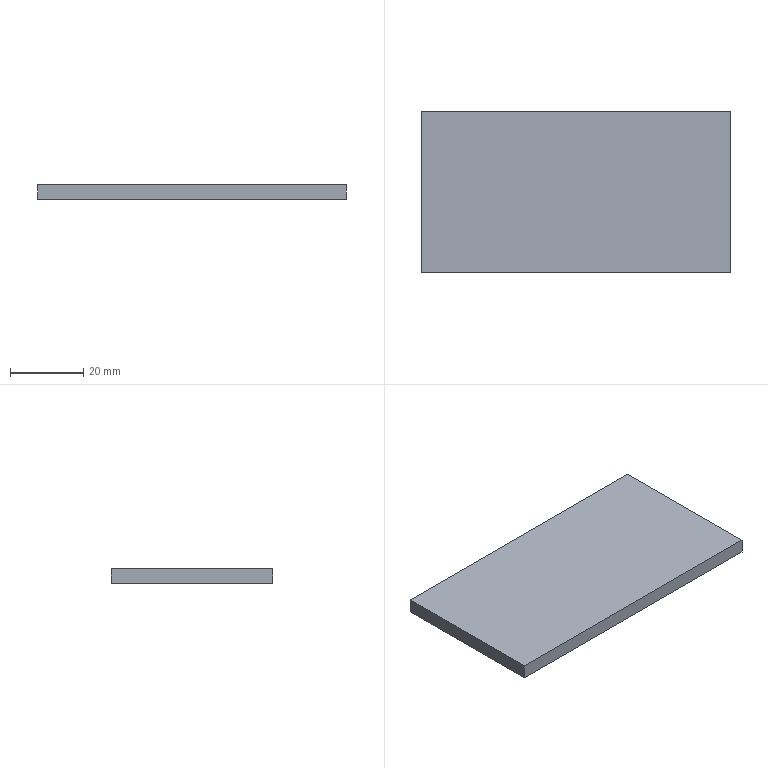Component | NX | BASE_PLATE | 1 solid | 6 faces | box 84 x 44 x 4 mm | volume 14784 mm3 | plane 6
STEP:
#1=CARTESIAN_POINT('',(0.,0.,0.));
#2=DIRECTION('',(0.,0.,1.));
#3=DIRECTION('',(1.,0.,0.));
#4=AXIS2_PLACEMENT_3D('',#1,#2,#3);
#5=CARTESIAN_POINT('',(-44.,24.,0.));
#6=VERTEX_POINT('',#5);
#7=CARTESIAN_POINT('',(-44.,-20.,0.));
#8=VERTEX_POINT('',#7);
#9=CARTESIAN_POINT('',(-44.,20.,0.));
#10=DIRECTION('',(0.,-1.,0.));
#11=VECTOR('',#10,1.);
#12=LINE('',#9,#11);
#13=CARTESIAN_POINT('',(-44.,20.,4.));
#14=DIRECTION('',(1.,0.,0.));
#15=DIRECTION('',(0.,0.,-1.));
#16=AXIS2_PLACEMENT_3D('',#13,#14,#15);
#17=PLANE('',#16);
#18=CARTESIAN_POINT('',(4.,0.));
#19=DIRECTION('',(0.,-1.));
#20=VECTOR('',#19,1.);
#21=LINE('',#18,#20);
#22=(GEOMETRIC_REPRESENTATION_CONTEXT(2)PARAMETRIC_REPRESENTATION_CONTEXT()REPRESENTATION_CONTEXT('',''));
#23=DEFINITIONAL_REPRESENTATION('',(#21),#22);
#24=PCURVE('',#17,#23);
#25=CARTESIAN_POINT('',(0.,0.,0.));
#26=DIRECTION('',(0.,0.,1.));
#27=DIRECTION('',(1.,0.,0.));
#28=AXIS2_PLACEMENT_3D('',#25,#26,#27);
#29=PLANE('',#28);
#30=CARTESIAN_POINT('',(-44.,20.));
#31=DIRECTION('',(0.,-1.));
#32=VECTOR('',#31,1.);
#33=LINE('',#30,#32);
#34=(GEOMETRIC_REPRESENTATION_CONTEXT(2)PARAMETRIC_REPRESENTATION_CONTEXT()REPRESENTATION_CONTEXT('',''));
#35=DEFINITIONAL_REPRESENTATION('',(#33),#34);
#36=PCURVE('',#29,#35);
#37=SURFACE_CURVE('',#12,(#24,#36),.PCURVE_S1.);
#38=EDGE_CURVE('',#6,#8,#37,.T.);
#39=ORIENTED_EDGE('',*,*,#38,.T.);
#40=CARTESIAN_POINT('',(-44.,-20.,4.));
#41=VERTEX_POINT('',#40);
#42=CARTESIAN_POINT('',(-44.,-20.,4.));
#43=DIRECTION('',(0.,0.,-1.));
#44=VECTOR('',#43,1.);
#45=LINE('',#42,#44);
#46=CARTESIAN_POINT('',(0.,-40.));
#47=DIRECTION('',(1.,0.));
#48=VECTOR('',#47,1.);
#49=LINE('',#46,#48);
#50=(GEOMETRIC_REPRESENTATION_CONTEXT(2)PARAMETRIC_REPRESENTATION_CONTEXT()REPRESENTATION_CONTEXT('',''));
#51=DEFINITIONAL_REPRESENTATION('',(#49),#50);
#52=PCURVE('',#17,#51);
#53=CARTESIAN_POINT('',(-40.,-20.,4.));
#54=DIRECTION('',(-0.,1.,0.));
#55=DIRECTION('',(-1.,-0.,0.));
#56=AXIS2_PLACEMENT_3D('',#53,#54,#55);
#57=PLANE('',#56);
#58=CARTESIAN_POINT('',(4.,0.));
#59=DIRECTION('',(0.,-1.));
#60=VECTOR('',#59,1.);
#61=LINE('',#58,#60);
#62=(GEOMETRIC_REPRESENTATION_CONTEXT(2)PARAMETRIC_REPRESENTATION_CONTEXT()REPRESENTATION_CONTEXT('',''));
#63=DEFINITIONAL_REPRESENTATION('',(#61),#62);
#64=PCURVE('',#57,#63);
#65=SURFACE_CURVE('',#45,(#52,#64),.PCURVE_S1.);
#66=EDGE_CURVE('',#41,#8,#65,.T.);
#67=ORIENTED_EDGE('',*,*,#66,.F.);
#68=CARTESIAN_POINT('',(-44.,24.,4.));
#69=VERTEX_POINT('',#68);
#70=CARTESIAN_POINT('',(-44.,20.,4.));
#71=DIRECTION('',(0.,-1.,0.));
#72=VECTOR('',#71,1.);
#73=LINE('',#70,#72);
#74=CARTESIAN_POINT('',(0.,0.));
#75=DIRECTION('',(0.,-1.));
#76=VECTOR('',#75,1.);
#77=LINE('',#74,#76);
#78=(GEOMETRIC_REPRESENTATION_CONTEXT(2)PARAMETRIC_REPRESENTATION_CONTEXT()REPRESENTATION_CONTEXT('',''));
#79=DEFINITIONAL_REPRESENTATION('',(#77),#78);
#80=PCURVE('',#17,#79);
#81=CARTESIAN_POINT('',(0.,0.,4.));
#82=DIRECTION('',(0.,0.,1.));
#83=DIRECTION('',(1.,0.,0.));
#84=AXIS2_PLACEMENT_3D('',#81,#82,#83);
#85=PLANE('',#84);
#86=CARTESIAN_POINT('',(-44.,20.));
#87=DIRECTION('',(0.,-1.));
#88=VECTOR('',#87,1.);
#89=LINE('',#86,#88);
#90=(GEOMETRIC_REPRESENTATION_CONTEXT(2)PARAMETRIC_REPRESENTATION_CONTEXT()REPRESENTATION_CONTEXT('',''));
#91=DEFINITIONAL_REPRESENTATION('',(#89),#90);
#92=PCURVE('',#85,#91);
#93=SURFACE_CURVE('',#73,(#80,#92),.PCURVE_S1.);
#94=EDGE_CURVE('',#69,#41,#93,.T.);
#95=ORIENTED_EDGE('',*,*,#94,.F.);
#96=CARTESIAN_POINT('',(-44.,24.,4.));
#97=DIRECTION('',(0.,0.,-1.));
#98=VECTOR('',#97,1.);
#99=LINE('',#96,#98);
#100=CARTESIAN_POINT('',(0.,4.));
#101=DIRECTION('',(1.,0.));
#102=VECTOR('',#101,1.);
#103=LINE('',#100,#102);
#104=(GEOMETRIC_REPRESENTATION_CONTEXT(2)PARAMETRIC_REPRESENTATION_CONTEXT()REPRESENTATION_CONTEXT('',''));
#105=DEFINITIONAL_REPRESENTATION('',(#103),#104);
#106=PCURVE('',#17,#105);
#107=CARTESIAN_POINT('',(40.,24.,4.));
#108=DIRECTION('',(-0.,-1.,0.));
#109=DIRECTION('',(1.,-0.,0.));
#110=AXIS2_PLACEMENT_3D('',#107,#108,#109);
#111=PLANE('',#110);
#112=CARTESIAN_POINT('',(-84.,0.));
#113=DIRECTION('',(0.,-1.));
#114=VECTOR('',#113,1.);
#115=LINE('',#112,#114);
#116=(GEOMETRIC_REPRESENTATION_CONTEXT(2)PARAMETRIC_REPRESENTATION_CONTEXT()REPRESENTATION_CONTEXT('',''));
#117=DEFINITIONAL_REPRESENTATION('',(#115),#116);
#118=PCURVE('',#111,#117);
#119=SURFACE_CURVE('',#99,(#106,#118),.PCURVE_S1.);
#120=EDGE_CURVE('',#69,#6,#119,.T.);
#121=ORIENTED_EDGE('',*,*,#120,.T.);
#122=EDGE_LOOP('',(#39,#67,#95,#121));
#123=FACE_BOUND('',#122,.T.);
#124=ADVANCED_FACE('',(#123),#17,.F.);
#125=CARTESIAN_POINT('',(40.,-20.,0.));
#126=VERTEX_POINT('',#125);
#127=CARTESIAN_POINT('',(-40.,-20.,0.));
#128=DIRECTION('',(1.,0.,0.));
#129=VECTOR('',#128,1.);
#130=LINE('',#127,#129);
#131=CARTESIAN_POINT('',(0.,-4.));
#132=DIRECTION('',(-1.,0.));
#133=VECTOR('',#132,1.);
#134=LINE('',#131,#133);
#135=(GEOMETRIC_REPRESENTATION_CONTEXT(2)PARAMETRIC_REPRESENTATION_CONTEXT()REPRESENTATION_CONTEXT('',''));
#136=DEFINITIONAL_REPRESENTATION('',(#134),#135);
#137=PCURVE('',#57,#136);
#138=CARTESIAN_POINT('',(-40.,-20.));
#139=DIRECTION('',(1.,0.));
#140=VECTOR('',#139,1.);
#141=LINE('',#138,#140);
#142=(GEOMETRIC_REPRESENTATION_CONTEXT(2)PARAMETRIC_REPRESENTATION_CONTEXT()REPRESENTATION_CONTEXT('',''));
#143=DEFINITIONAL_REPRESENTATION('',(#141),#142);
#144=PCURVE('',#29,#143);
#145=SURFACE_CURVE('',#130,(#137,#144),.PCURVE_S1.);
#146=EDGE_CURVE('',#8,#126,#145,.T.);
#147=ORIENTED_EDGE('',*,*,#146,.T.);
#148=CARTESIAN_POINT('',(40.,-20.,4.));
#149=VERTEX_POINT('',#148);
#150=CARTESIAN_POINT('',(40.,-20.,4.));
#151=DIRECTION('',(0.,0.,-1.));
#152=VECTOR('',#151,1.);
#153=LINE('',#150,#152);
#154=CARTESIAN_POINT('',(-80.,0.));
#155=DIRECTION('',(0.,-1.));
#156=VECTOR('',#155,1.);
#157=LINE('',#154,#156);
#158=(GEOMETRIC_REPRESENTATION_CONTEXT(2)PARAMETRIC_REPRESENTATION_CONTEXT()REPRESENTATION_CONTEXT('',''));
#159=DEFINITIONAL_REPRESENTATION('',(#157),#158);
#160=PCURVE('',#57,#159);
#161=CARTESIAN_POINT('',(40.,-20.,4.));
#162=DIRECTION('',(-1.,0.,0.));
#163=DIRECTION('',(0.,0.,1.));
#164=AXIS2_PLACEMENT_3D('',#161,#162,#163);
#165=PLANE('',#164);
#166=CARTESIAN_POINT('',(0.,0.));
#167=DIRECTION('',(-1.,0.));
#168=VECTOR('',#167,1.);
#169=LINE('',#166,#168);
#170=(GEOMETRIC_REPRESENTATION_CONTEXT(2)PARAMETRIC_REPRESENTATION_CONTEXT()REPRESENTATION_CONTEXT('',''));
#171=DEFINITIONAL_REPRESENTATION('',(#169),#170);
#172=PCURVE('',#165,#171);
#173=SURFACE_CURVE('',#153,(#160,#172),.PCURVE_S1.);
#174=EDGE_CURVE('',#149,#126,#173,.T.);
#175=ORIENTED_EDGE('',*,*,#174,.F.);
#176=CARTESIAN_POINT('',(-40.,-20.,4.));
#177=DIRECTION('',(1.,0.,0.));
#178=VECTOR('',#177,1.);
#179=LINE('',#176,#178);
#180=CARTESIAN_POINT('',(0.,0.));
#181=DIRECTION('',(-1.,0.));
#182=VECTOR('',#181,1.);
#183=LINE('',#180,#182);
#184=(GEOMETRIC_REPRESENTATION_CONTEXT(2)PARAMETRIC_REPRESENTATION_CONTEXT()REPRESENTATION_CONTEXT('',''));
#185=DEFINITIONAL_REPRESENTATION('',(#183),#184);
#186=PCURVE('',#57,#185);
#187=CARTESIAN_POINT('',(-40.,-20.));
#188=DIRECTION('',(1.,0.));
#189=VECTOR('',#188,1.);
#190=LINE('',#187,#189);
#191=(GEOMETRIC_REPRESENTATION_CONTEXT(2)PARAMETRIC_REPRESENTATION_CONTEXT()REPRESENTATION_CONTEXT('',''));
#192=DEFINITIONAL_REPRESENTATION('',(#190),#191);
#193=PCURVE('',#85,#192);
#194=SURFACE_CURVE('',#179,(#186,#193),.PCURVE_S1.);
#195=EDGE_CURVE('',#41,#149,#194,.T.);
#196=ORIENTED_EDGE('',*,*,#195,.F.);
#197=ORIENTED_EDGE('',*,*,#66,.T.);
#198=EDGE_LOOP('',(#147,#175,#196,#197));
#199=FACE_BOUND('',#198,.T.);
#200=ADVANCED_FACE('',(#199),#57,.F.);
#201=CARTESIAN_POINT('',(40.,24.,0.));
#202=VERTEX_POINT('',#201);
#203=CARTESIAN_POINT('',(40.,-20.,0.));
#204=DIRECTION('',(0.,1.,0.));
#205=VECTOR('',#204,1.);
#206=LINE('',#203,#205);
#207=CARTESIAN_POINT('',(-4.,0.));
#208=DIRECTION('',(0.,1.));
#209=VECTOR('',#208,1.);
#210=LINE('',#207,#209);
#211=(GEOMETRIC_REPRESENTATION_CONTEXT(2)PARAMETRIC_REPRESENTATION_CONTEXT()REPRESENTATION_CONTEXT('',''));
#212=DEFINITIONAL_REPRESENTATION('',(#210),#211);
#213=PCURVE('',#165,#212);
#214=CARTESIAN_POINT('',(40.,-20.));
#215=DIRECTION('',(0.,1.));
#216=VECTOR('',#215,1.);
#217=LINE('',#214,#216);
#218=(GEOMETRIC_REPRESENTATION_CONTEXT(2)PARAMETRIC_REPRESENTATION_CONTEXT()REPRESENTATION_CONTEXT('',''));
#219=DEFINITIONAL_REPRESENTATION('',(#217),#218);
#220=PCURVE('',#29,#219);
#221=SURFACE_CURVE('',#206,(#213,#220),.PCURVE_S1.);
#222=EDGE_CURVE('',#126,#202,#221,.T.);
#223=ORIENTED_EDGE('',*,*,#222,.T.);
#224=CARTESIAN_POINT('',(40.,24.,4.));
#225=VERTEX_POINT('',#224);
#226=CARTESIAN_POINT('',(40.,24.,4.));
#227=DIRECTION('',(0.,0.,-1.));
#228=VECTOR('',#227,1.);
#229=LINE('',#226,#228);
#230=CARTESIAN_POINT('',(0.,44.));
#231=DIRECTION('',(-1.,0.));
#232=VECTOR('',#231,1.);
#233=LINE('',#230,#232);
#234=(GEOMETRIC_REPRESENTATION_CONTEXT(2)PARAMETRIC_REPRESENTATION_CONTEXT()REPRESENTATION_CONTEXT('',''));
#235=DEFINITIONAL_REPRESENTATION('',(#233),#234);
#236=PCURVE('',#165,#235);
#237=CARTESIAN_POINT('',(0.,0.));
#238=DIRECTION('',(0.,-1.));
#239=VECTOR('',#238,1.);
#240=LINE('',#237,#239);
#241=(GEOMETRIC_REPRESENTATION_CONTEXT(2)PARAMETRIC_REPRESENTATION_CONTEXT()REPRESENTATION_CONTEXT('',''));
#242=DEFINITIONAL_REPRESENTATION('',(#240),#241);
#243=PCURVE('',#111,#242);
#244=SURFACE_CURVE('',#229,(#236,#243),.PCURVE_S1.);
#245=EDGE_CURVE('',#225,#202,#244,.T.);
#246=ORIENTED_EDGE('',*,*,#245,.F.);
#247=CARTESIAN_POINT('',(40.,-20.,4.));
#248=DIRECTION('',(0.,1.,0.));
#249=VECTOR('',#248,1.);
#250=LINE('',#247,#249);
#251=CARTESIAN_POINT('',(0.,0.));
#252=DIRECTION('',(0.,1.));
#253=VECTOR('',#252,1.);
#254=LINE('',#251,#253);
#255=(GEOMETRIC_REPRESENTATION_CONTEXT(2)PARAMETRIC_REPRESENTATION_CONTEXT()REPRESENTATION_CONTEXT('',''));
#256=DEFINITIONAL_REPRESENTATION('',(#254),#255);
#257=PCURVE('',#165,#256);
#258=CARTESIAN_POINT('',(40.,-20.));
#259=DIRECTION('',(0.,1.));
#260=VECTOR('',#259,1.);
#261=LINE('',#258,#260);
#262=(GEOMETRIC_REPRESENTATION_CONTEXT(2)PARAMETRIC_REPRESENTATION_CONTEXT()REPRESENTATION_CONTEXT('',''));
#263=DEFINITIONAL_REPRESENTATION('',(#261),#262);
#264=PCURVE('',#85,#263);
#265=SURFACE_CURVE('',#250,(#257,#264),.PCURVE_S1.);
#266=EDGE_CURVE('',#149,#225,#265,.T.);
#267=ORIENTED_EDGE('',*,*,#266,.F.);
#268=ORIENTED_EDGE('',*,*,#174,.T.);
#269=EDGE_LOOP('',(#223,#246,#267,#268));
#270=FACE_BOUND('',#269,.T.);
#271=ADVANCED_FACE('',(#270),#165,.F.);
#272=CARTESIAN_POINT('',(40.,24.,0.));
#273=DIRECTION('',(-1.,0.,0.));
#274=VECTOR('',#273,1.);
#275=LINE('',#272,#274);
#276=CARTESIAN_POINT('',(0.,-4.));
#277=DIRECTION('',(-1.,0.));
#278=VECTOR('',#277,1.);
#279=LINE('',#276,#278);
#280=(GEOMETRIC_REPRESENTATION_CONTEXT(2)PARAMETRIC_REPRESENTATION_CONTEXT()REPRESENTATION_CONTEXT('',''));
#281=DEFINITIONAL_REPRESENTATION('',(#279),#280);
#282=PCURVE('',#111,#281);
#283=CARTESIAN_POINT('',(40.,24.));
#284=DIRECTION('',(-1.,0.));
#285=VECTOR('',#284,1.);
#286=LINE('',#283,#285);
#287=(GEOMETRIC_REPRESENTATION_CONTEXT(2)PARAMETRIC_REPRESENTATION_CONTEXT()REPRESENTATION_CONTEXT('',''));
#288=DEFINITIONAL_REPRESENTATION('',(#286),#287);
#289=PCURVE('',#29,#288);
#290=SURFACE_CURVE('',#275,(#282,#289),.PCURVE_S1.);
#291=EDGE_CURVE('',#202,#6,#290,.T.);
#292=ORIENTED_EDGE('',*,*,#291,.T.);
#293=ORIENTED_EDGE('',*,*,#120,.F.);
#294=CARTESIAN_POINT('',(40.,24.,4.));
#295=DIRECTION('',(-1.,0.,0.));
#296=VECTOR('',#295,1.);
#297=LINE('',#294,#296);
#298=CARTESIAN_POINT('',(0.,0.));
#299=DIRECTION('',(-1.,0.));
#300=VECTOR('',#299,1.);
#301=LINE('',#298,#300);
#302=(GEOMETRIC_REPRESENTATION_CONTEXT(2)PARAMETRIC_REPRESENTATION_CONTEXT()REPRESENTATION_CONTEXT('',''));
#303=DEFINITIONAL_REPRESENTATION('',(#301),#302);
#304=PCURVE('',#111,#303);
#305=CARTESIAN_POINT('',(40.,24.));
#306=DIRECTION('',(-1.,0.));
#307=VECTOR('',#306,1.);
#308=LINE('',#305,#307);
#309=(GEOMETRIC_REPRESENTATION_CONTEXT(2)PARAMETRIC_REPRESENTATION_CONTEXT()REPRESENTATION_CONTEXT('',''));
#310=DEFINITIONAL_REPRESENTATION('',(#308),#309);
#311=PCURVE('',#85,#310);
#312=SURFACE_CURVE('',#297,(#304,#311),.PCURVE_S1.);
#313=EDGE_CURVE('',#225,#69,#312,.T.);
#314=ORIENTED_EDGE('',*,*,#313,.F.);
#315=ORIENTED_EDGE('',*,*,#245,.T.);
#316=EDGE_LOOP('',(#292,#293,#314,#315));
#317=FACE_BOUND('',#316,.T.);
#318=ADVANCED_FACE('',(#317),#111,.F.);
#319=ORIENTED_EDGE('',*,*,#94,.T.);
#320=ORIENTED_EDGE('',*,*,#195,.T.);
#321=ORIENTED_EDGE('',*,*,#266,.T.);
#322=ORIENTED_EDGE('',*,*,#313,.T.);
#323=EDGE_LOOP('',(#319,#320,#321,#322));
#324=FACE_BOUND('',#323,.T.);
#325=ADVANCED_FACE('',(#324),#85,.T.);
#326=ORIENTED_EDGE('',*,*,#38,.F.);
#327=ORIENTED_EDGE('',*,*,#291,.F.);
#328=ORIENTED_EDGE('',*,*,#222,.F.);
#329=ORIENTED_EDGE('',*,*,#146,.F.);
#330=EDGE_LOOP('',(#326,#327,#328,#329));
#331=FACE_BOUND('',#330,.T.);
#332=ADVANCED_FACE('',(#331),#29,.F.);
#333=CLOSED_SHELL('',(#124,#200,#271,#318,#325,#332));
#334=MANIFOLD_SOLID_BREP('',#333);
#335=(LENGTH_UNIT()NAMED_UNIT(*)SI_UNIT(.MILLI.,.METRE.));
#336=UNCERTAINTY_MEASURE_WITH_UNIT(LENGTH_MEASURE(0.0000001),#335,'','');
#337=(NAMED_UNIT(*)PLANE_ANGLE_UNIT()SI_UNIT($,.RADIAN.));
#338=(NAMED_UNIT(*)SI_UNIT($,.STERADIAN.)SOLID_ANGLE_UNIT());
#339=(GEOMETRIC_REPRESENTATION_CONTEXT(3)GLOBAL_UNCERTAINTY_ASSIGNED_CONTEXT((#336))GLOBAL_UNIT_ASSIGNED_CONTEXT((#335,#337,#338))REPRESENTATION_CONTEXT('',''));
#340=ADVANCED_BREP_SHAPE_REPRESENTATION('',(#4,#334),#339);